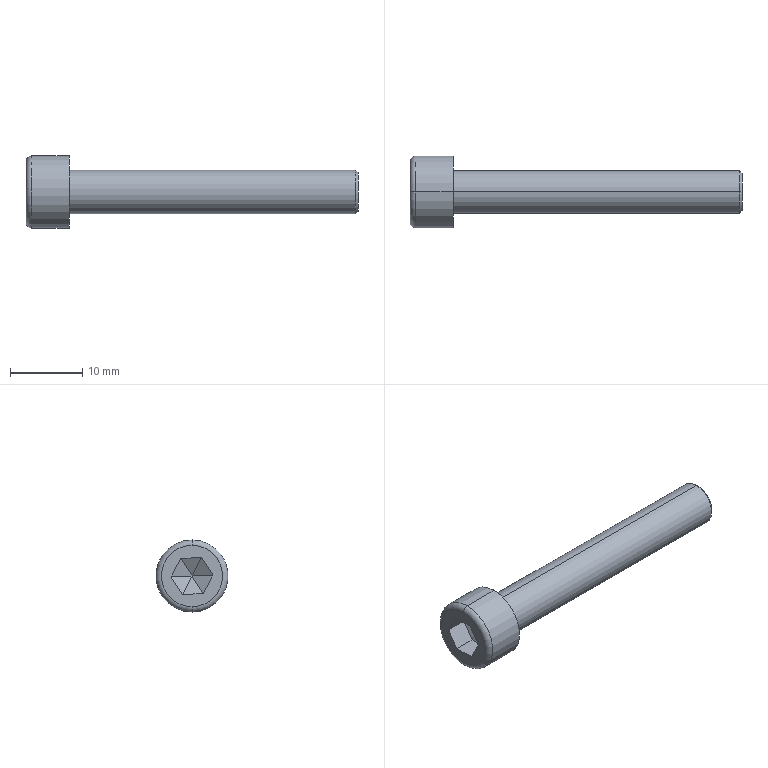Component | SolidWorks | 170423A4-ConveyorBeltIdlerAssembly1-1_170423A4-M6X40StainlessSteelCupHeadHexSocket-1 | 1 solid | 23 faces | box 46 x 10 x 10 mm | volume 1522 mm3 | plane 15 | cylinder 4 | cone 2 | torus 2 | commonest cylinder face diameters 6 x2 10 x2
STEP:
#1=CARTESIAN_POINT('',(-0.679,-3.771,17.671));
#2=VERTEX_POINT('',#1);
#3=CARTESIAN_POINT('',(-0.679,-3.771,17.88));
#4=VERTEX_POINT('',#3);
#5=CARTESIAN_POINT('',(-0.679,-3.771,17.776));
#6=DIRECTION('',(1.,0.,0.));
#7=DIRECTION('',(0.,0.,-1.));
#8=AXIS2_PLACEMENT_3D('',#5,#6,#7);
#9=CIRCLE('',#8,0.1043);
#10=EDGE_CURVE('',#2,#4,#9,.T.);
#11=ORIENTED_EDGE('',*,*,#10,.F.);
#12=CARTESIAN_POINT('',(-0.6928,-3.771,17.657));
#13=VERTEX_POINT('',#12);
#14=CARTESIAN_POINT('',(-0.679,-3.771,17.671));
#15=DIRECTION('',(-0.7071,0.,-0.7071));
#16=VECTOR('',#15,39.37);
#17=LINE('',#14,#16);
#18=EDGE_CURVE('',#2,#13,#17,.T.);
#19=ORIENTED_EDGE('',*,*,#18,.T.);
#20=CARTESIAN_POINT('',(-0.6928,-3.771,17.894));
#21=VERTEX_POINT('',#20);
#22=CARTESIAN_POINT('',(-0.6928,-3.771,17.776));
#23=DIRECTION('',(-1.,0.,0.));
#24=DIRECTION('',(0.,0.,-1.));
#25=AXIS2_PLACEMENT_3D('',#22,#23,#24);
#26=CIRCLE('',#25,0.1181);
#27=EDGE_CURVE('',#21,#13,#26,.T.);
#28=ORIENTED_EDGE('',*,*,#27,.F.);
#29=CARTESIAN_POINT('',(-0.679,-3.771,17.88));
#30=DIRECTION('',(-0.7071,0.,0.7071));
#31=VECTOR('',#30,39.37);
#32=LINE('',#29,#31);
#33=EDGE_CURVE('',#4,#21,#32,.T.);
#34=ORIENTED_EDGE('',*,*,#33,.F.);
#35=EDGE_LOOP('',(#11,#19,#28,#34));
#36=FACE_OUTER_BOUND('',#35,.T.);
#37=CARTESIAN_POINT('',(-0.679,-3.771,17.776));
#38=DIRECTION('',(-1.,0.,0.));
#39=DIRECTION('',(0.,0.,1.));
#40=AXIS2_PLACEMENT_3D('',#37,#38,#39);
#41=CONICAL_SURFACE('',#40,0.1043,0.7854);
#42=ADVANCED_FACE('',(#36),#41,.T.);
#43=CARTESIAN_POINT('',(-2.46,-3.771,17.579));
#44=VERTEX_POINT('',#43);
#45=CARTESIAN_POINT('',(-2.46,-3.771,17.972));
#46=VERTEX_POINT('',#45);
#47=CARTESIAN_POINT('',(-2.46,-3.771,17.776));
#48=DIRECTION('',(1.,0.,0.));
#49=DIRECTION('',(0.,0.,1.));
#50=AXIS2_PLACEMENT_3D('',#47,#48,#49);
#51=CIRCLE('',#50,0.1969);
#52=EDGE_CURVE('',#44,#46,#51,.T.);
#53=ORIENTED_EDGE('',*,*,#52,.F.);
#54=CARTESIAN_POINT('',(-2.49,-3.771,17.608));
#55=VERTEX_POINT('',#54);
#56=CARTESIAN_POINT('',(-2.46,-3.771,17.608));
#57=DIRECTION('',(0.,1.,0.));
#58=DIRECTION('',(0.,0.,1.));
#59=AXIS2_PLACEMENT_3D('',#56,#57,#58);
#60=CIRCLE('',#59,0.02953);
#61=EDGE_CURVE('',#44,#55,#60,.T.);
#62=ORIENTED_EDGE('',*,*,#61,.T.);
#63=CARTESIAN_POINT('',(-2.49,-3.771,17.943));
#64=VERTEX_POINT('',#63);
#65=CARTESIAN_POINT('',(-2.49,-3.771,17.776));
#66=DIRECTION('',(-1.,0.,0.));
#67=DIRECTION('',(0.,0.,1.));
#68=AXIS2_PLACEMENT_3D('',#65,#66,#67);
#69=CIRCLE('',#68,0.1673);
#70=EDGE_CURVE('',#64,#55,#69,.T.);
#71=ORIENTED_EDGE('',*,*,#70,.F.);
#72=CARTESIAN_POINT('',(-2.46,-3.771,17.943));
#73=DIRECTION('',(0.,-1.,0.));
#74=DIRECTION('',(0.,0.,-1.));
#75=AXIS2_PLACEMENT_3D('',#72,#73,#74);
#76=CIRCLE('',#75,0.02953);
#77=EDGE_CURVE('',#46,#64,#76,.T.);
#78=ORIENTED_EDGE('',*,*,#77,.F.);
#79=EDGE_LOOP('',(#53,#62,#71,#78));
#80=FACE_OUTER_BOUND('',#79,.T.);
#81=CARTESIAN_POINT('',(-2.46,-3.771,17.776));
#82=DIRECTION('',(-1.,0.,0.));
#83=DIRECTION('',(0.,0.,1.));
#84=AXIS2_PLACEMENT_3D('',#81,#82,#83);
#85=TOROIDAL_SURFACE('',#84,0.1673,0.02953);
#86=ADVANCED_FACE('',(#80),#85,.T.);
#87=ORIENTED_EDGE('',*,*,#27,.T.);
#88=CARTESIAN_POINT('',(-2.254,-3.771,17.657));
#89=VERTEX_POINT('',#88);
#90=CARTESIAN_POINT('',(-0.679,-3.771,17.657));
#91=DIRECTION('',(-1.,0.,0.));
#92=VECTOR('',#91,39.37);
#93=LINE('',#90,#92);
#94=EDGE_CURVE('',#13,#89,#93,.T.);
#95=ORIENTED_EDGE('',*,*,#94,.T.);
#96=CARTESIAN_POINT('',(-2.254,-3.771,17.894));
#97=VERTEX_POINT('',#96);
#98=CARTESIAN_POINT('',(-2.254,-3.771,17.776));
#99=DIRECTION('',(1.,0.,0.));
#100=DIRECTION('',(0.,0.,1.));
#101=AXIS2_PLACEMENT_3D('',#98,#99,#100);
#102=CIRCLE('',#101,0.1181);
#103=EDGE_CURVE('',#89,#97,#102,.T.);
#104=ORIENTED_EDGE('',*,*,#103,.T.);
#105=CARTESIAN_POINT('',(-0.679,-3.771,17.894));
#106=DIRECTION('',(-1.,0.,0.));
#107=VECTOR('',#106,39.37);
#108=LINE('',#105,#107);
#109=EDGE_CURVE('',#21,#97,#108,.T.);
#110=ORIENTED_EDGE('',*,*,#109,.F.);
#111=EDGE_LOOP('',(#87,#95,#104,#110));
#112=FACE_OUTER_BOUND('',#111,.T.);
#113=CARTESIAN_POINT('',(-0.679,-3.771,17.776));
#114=DIRECTION('',(-1.,0.,0.));
#115=DIRECTION('',(0.,0.,1.));
#116=AXIS2_PLACEMENT_3D('',#113,#114,#115);
#117=CYLINDRICAL_SURFACE('',#116,0.1181);
#118=ADVANCED_FACE('',(#112),#117,.T.);
#119=ORIENTED_EDGE('',*,*,#52,.T.);
#120=CARTESIAN_POINT('',(-2.254,-3.771,17.972));
#121=VERTEX_POINT('',#120);
#122=CARTESIAN_POINT('',(-2.49,-3.771,17.972));
#123=DIRECTION('',(1.,0.,0.));
#124=VECTOR('',#123,39.37);
#125=LINE('',#122,#124);
#126=EDGE_CURVE('',#46,#121,#125,.T.);
#127=ORIENTED_EDGE('',*,*,#126,.T.);
#128=CARTESIAN_POINT('',(-2.254,-3.771,17.579));
#129=VERTEX_POINT('',#128);
#130=CARTESIAN_POINT('',(-2.254,-3.771,17.776));
#131=DIRECTION('',(-1.,0.,0.));
#132=DIRECTION('',(0.,0.,1.));
#133=AXIS2_PLACEMENT_3D('',#130,#131,#132);
#134=CIRCLE('',#133,0.1969);
#135=EDGE_CURVE('',#121,#129,#134,.T.);
#136=ORIENTED_EDGE('',*,*,#135,.T.);
#137=CARTESIAN_POINT('',(-2.49,-3.771,17.579));
#138=DIRECTION('',(1.,0.,0.));
#139=VECTOR('',#138,39.37);
#140=LINE('',#137,#139);
#141=EDGE_CURVE('',#44,#129,#140,.T.);
#142=ORIENTED_EDGE('',*,*,#141,.F.);
#143=EDGE_LOOP('',(#119,#127,#136,#142));
#144=FACE_OUTER_BOUND('',#143,.T.);
#145=CARTESIAN_POINT('',(-2.49,-3.771,17.776));
#146=DIRECTION('',(1.,0.,0.));
#147=DIRECTION('',(0.,0.,-1.));
#148=AXIS2_PLACEMENT_3D('',#145,#146,#147);
#149=CYLINDRICAL_SURFACE('',#148,0.1969);
#150=ADVANCED_FACE('',(#144),#149,.T.);
#151=CARTESIAN_POINT('',(-2.254,-3.771,17.776));
#152=DIRECTION('',(-1.,0.,0.));
#153=DIRECTION('',(0.,0.,1.));
#154=AXIS2_PLACEMENT_3D('',#151,#152,#153);
#155=CIRCLE('',#154,0.1969);
#156=EDGE_CURVE('',#129,#121,#155,.T.);
#157=ORIENTED_EDGE('',*,*,#156,.F.);
#158=ORIENTED_EDGE('',*,*,#135,.F.);
#159=EDGE_LOOP('',(#157,#158));
#160=FACE_OUTER_BOUND('',#159,.T.);
#161=CARTESIAN_POINT('',(-2.254,-3.771,17.776));
#162=DIRECTION('',(1.,0.,0.));
#163=DIRECTION('',(0.,0.,1.));
#164=AXIS2_PLACEMENT_3D('',#161,#162,#163);
#165=CIRCLE('',#164,0.1181);
#166=EDGE_CURVE('',#97,#89,#165,.T.);
#167=ORIENTED_EDGE('',*,*,#166,.F.);
#168=ORIENTED_EDGE('',*,*,#103,.F.);
#169=EDGE_LOOP('',(#167,#168));
#170=FACE_BOUND('',#169,.T.);
#171=CARTESIAN_POINT('',(-2.254,-3.771,17.776));
#172=DIRECTION('',(-1.,0.,0.));
#173=DIRECTION('',(0.,0.,1.));
#174=AXIS2_PLACEMENT_3D('',#171,#172,#173);
#175=PLANE('',#174);
#176=ADVANCED_FACE('',(#160,#170),#175,.F.);
#177=ORIENTED_EDGE('',*,*,#126,.F.);
#178=CARTESIAN_POINT('',(-2.46,-3.771,17.776));
#179=DIRECTION('',(1.,0.,0.));
#180=DIRECTION('',(0.,0.,1.));
#181=AXIS2_PLACEMENT_3D('',#178,#179,#180);
#182=CIRCLE('',#181,0.1969);
#183=EDGE_CURVE('',#46,#44,#182,.T.);
#184=ORIENTED_EDGE('',*,*,#183,.T.);
#185=ORIENTED_EDGE('',*,*,#141,.T.);
#186=ORIENTED_EDGE('',*,*,#156,.T.);
#187=EDGE_LOOP('',(#177,#184,#185,#186));
#188=FACE_OUTER_BOUND('',#187,.T.);
#189=CARTESIAN_POINT('',(-2.49,-3.771,17.776));
#190=DIRECTION('',(1.,0.,0.));
#191=DIRECTION('',(0.,0.,-1.));
#192=AXIS2_PLACEMENT_3D('',#189,#190,#191);
#193=CYLINDRICAL_SURFACE('',#192,0.1969);
#194=ADVANCED_FACE('',(#188),#193,.T.);
#195=ORIENTED_EDGE('',*,*,#70,.T.);
#196=CARTESIAN_POINT('',(-2.49,-3.771,17.776));
#197=DIRECTION('',(-1.,0.,0.));
#198=DIRECTION('',(0.,0.,1.));
#199=AXIS2_PLACEMENT_3D('',#196,#197,#198);
#200=CIRCLE('',#199,0.1673);
#201=EDGE_CURVE('',#55,#64,#200,.T.);
#202=ORIENTED_EDGE('',*,*,#201,.T.);
#203=EDGE_LOOP('',(#195,#202));
#204=FACE_OUTER_BOUND('',#203,.T.);
#205=CARTESIAN_POINT('',(-2.49,-3.833,17.68));
#206=VERTEX_POINT('',#205);
#207=CARTESIAN_POINT('',(-2.49,-3.885,17.781));
#208=VERTEX_POINT('',#207);
#209=CARTESIAN_POINT('',(-2.49,-3.833,17.68));
#210=DIRECTION('',(0.,-0.4558,0.8901));
#211=VECTOR('',#210,39.37);
#212=LINE('',#209,#211);
#213=EDGE_CURVE('',#206,#208,#212,.T.);
#214=ORIENTED_EDGE('',*,*,#213,.F.);
#215=CARTESIAN_POINT('',(-2.49,-3.719,17.674));
#216=VERTEX_POINT('',#215);
#217=CARTESIAN_POINT('',(-2.49,-3.719,17.674));
#218=DIRECTION('',(0.,-0.9987,0.05033));
#219=VECTOR('',#218,39.37);
#220=LINE('',#217,#219);
#221=EDGE_CURVE('',#216,#206,#220,.T.);
#222=ORIENTED_EDGE('',*,*,#221,.F.);
#223=CARTESIAN_POINT('',(-2.49,-3.658,17.77));
#224=VERTEX_POINT('',#223);
#225=CARTESIAN_POINT('',(-2.49,-3.658,17.77));
#226=DIRECTION('',(0.,-0.543,-0.8398));
#227=VECTOR('',#226,39.37);
#228=LINE('',#225,#227);
#229=EDGE_CURVE('',#224,#216,#228,.T.);
#230=ORIENTED_EDGE('',*,*,#229,.F.);
#231=CARTESIAN_POINT('',(-2.49,-3.709,17.871));
#232=VERTEX_POINT('',#231);
#233=CARTESIAN_POINT('',(-2.49,-3.709,17.871));
#234=DIRECTION('',(0.,0.4558,-0.8901));
#235=VECTOR('',#234,39.37);
#236=LINE('',#233,#235);
#237=EDGE_CURVE('',#232,#224,#236,.T.);
#238=ORIENTED_EDGE('',*,*,#237,.F.);
#239=CARTESIAN_POINT('',(-2.49,-3.823,17.877));
#240=VERTEX_POINT('',#239);
#241=CARTESIAN_POINT('',(-2.49,-3.823,17.877));
#242=DIRECTION('',(0.,0.9987,-0.05033));
#243=VECTOR('',#242,39.37);
#244=LINE('',#241,#243);
#245=EDGE_CURVE('',#240,#232,#244,.T.);
#246=ORIENTED_EDGE('',*,*,#245,.F.);
#247=CARTESIAN_POINT('',(-2.49,-3.885,17.781));
#248=DIRECTION('',(0.,0.543,0.8398));
#249=VECTOR('',#248,39.37);
#250=LINE('',#247,#249);
#251=EDGE_CURVE('',#208,#240,#250,.T.);
#252=ORIENTED_EDGE('',*,*,#251,.F.);
#253=EDGE_LOOP('',(#214,#222,#230,#238,#246,#252));
#254=FACE_BOUND('',#253,.T.);
#255=CARTESIAN_POINT('',(-2.49,-3.771,17.776));
#256=DIRECTION('',(-1.,0.,0.));
#257=DIRECTION('',(0.,0.,1.));
#258=AXIS2_PLACEMENT_3D('',#255,#256,#257);
#259=PLANE('',#258);
#260=ADVANCED_FACE('',(#204,#254),#259,.T.);
#261=ORIENTED_EDGE('',*,*,#213,.T.);
#262=CARTESIAN_POINT('',(-2.372,-3.885,17.781));
#263=VERTEX_POINT('',#262);
#264=CARTESIAN_POINT('',(-2.372,-3.885,17.781));
#265=DIRECTION('',(-1.,0.,0.));
#266=VECTOR('',#265,39.37);
#267=LINE('',#264,#266);
#268=EDGE_CURVE('',#263,#208,#267,.T.);
#269=ORIENTED_EDGE('',*,*,#268,.F.);
#270=CARTESIAN_POINT('',(-2.372,-3.833,17.68));
#271=VERTEX_POINT('',#270);
#272=CARTESIAN_POINT('',(-2.372,-3.833,17.68));
#273=DIRECTION('',(0.,-0.4558,0.8901));
#274=VECTOR('',#273,39.37);
#275=LINE('',#272,#274);
#276=EDGE_CURVE('',#271,#263,#275,.T.);
#277=ORIENTED_EDGE('',*,*,#276,.F.);
#278=CARTESIAN_POINT('',(-2.372,-3.833,17.68));
#279=DIRECTION('',(-1.,0.,0.));
#280=VECTOR('',#279,39.37);
#281=LINE('',#278,#280);
#282=EDGE_CURVE('',#271,#206,#281,.T.);
#283=ORIENTED_EDGE('',*,*,#282,.T.);
#284=EDGE_LOOP('',(#261,#269,#277,#283));
#285=FACE_OUTER_BOUND('',#284,.T.);
#286=CARTESIAN_POINT('',(-2.372,-3.833,17.68));
#287=DIRECTION('',(0.,-0.8901,-0.4558));
#288=DIRECTION('',(0.,-0.4558,0.8901));
#289=AXIS2_PLACEMENT_3D('',#286,#287,#288);
#290=PLANE('',#289);
#291=ADVANCED_FACE('',(#285),#290,.F.);
#292=ORIENTED_EDGE('',*,*,#221,.T.);
#293=ORIENTED_EDGE('',*,*,#282,.F.);
#294=CARTESIAN_POINT('',(-2.372,-3.719,17.674));
#295=VERTEX_POINT('',#294);
#296=CARTESIAN_POINT('',(-2.372,-3.719,17.674));
#297=DIRECTION('',(0.,-0.9987,0.05033));
#298=VECTOR('',#297,39.37);
#299=LINE('',#296,#298);
#300=EDGE_CURVE('',#295,#271,#299,.T.);
#301=ORIENTED_EDGE('',*,*,#300,.F.);
#302=CARTESIAN_POINT('',(-2.372,-3.719,17.674));
#303=DIRECTION('',(-1.,0.,0.));
#304=VECTOR('',#303,39.37);
#305=LINE('',#302,#304);
#306=EDGE_CURVE('',#295,#216,#305,.T.);
#307=ORIENTED_EDGE('',*,*,#306,.T.);
#308=EDGE_LOOP('',(#292,#293,#301,#307));
#309=FACE_OUTER_BOUND('',#308,.T.);
#310=CARTESIAN_POINT('',(-2.372,-3.719,17.674));
#311=DIRECTION('',(0.,-0.05033,-0.9987));
#312=DIRECTION('',(0.,-0.9987,0.05033));
#313=AXIS2_PLACEMENT_3D('',#310,#311,#312);
#314=PLANE('',#313);
#315=ADVANCED_FACE('',(#309),#314,.F.);
#316=ORIENTED_EDGE('',*,*,#229,.T.);
#317=ORIENTED_EDGE('',*,*,#306,.F.);
#318=CARTESIAN_POINT('',(-2.372,-3.658,17.77));
#319=VERTEX_POINT('',#318);
#320=CARTESIAN_POINT('',(-2.372,-3.658,17.77));
#321=DIRECTION('',(0.,-0.543,-0.8398));
#322=VECTOR('',#321,39.37);
#323=LINE('',#320,#322);
#324=EDGE_CURVE('',#319,#295,#323,.T.);
#325=ORIENTED_EDGE('',*,*,#324,.F.);
#326=CARTESIAN_POINT('',(-2.372,-3.658,17.77));
#327=DIRECTION('',(-1.,0.,0.));
#328=VECTOR('',#327,39.37);
#329=LINE('',#326,#328);
#330=EDGE_CURVE('',#319,#224,#329,.T.);
#331=ORIENTED_EDGE('',*,*,#330,.T.);
#332=EDGE_LOOP('',(#316,#317,#325,#331));
#333=FACE_OUTER_BOUND('',#332,.T.);
#334=CARTESIAN_POINT('',(-2.372,-3.658,17.77));
#335=DIRECTION('',(0.,0.8398,-0.543));
#336=DIRECTION('',(0.,-0.543,-0.8398));
#337=AXIS2_PLACEMENT_3D('',#334,#335,#336);
#338=PLANE('',#337);
#339=ADVANCED_FACE('',(#333),#338,.F.);
#340=ORIENTED_EDGE('',*,*,#237,.T.);
#341=ORIENTED_EDGE('',*,*,#330,.F.);
#342=CARTESIAN_POINT('',(-2.372,-3.709,17.871));
#343=VERTEX_POINT('',#342);
#344=CARTESIAN_POINT('',(-2.372,-3.709,17.871));
#345=DIRECTION('',(0.,0.4558,-0.8901));
#346=VECTOR('',#345,39.37);
#347=LINE('',#344,#346);
#348=EDGE_CURVE('',#343,#319,#347,.T.);
#349=ORIENTED_EDGE('',*,*,#348,.F.);
#350=CARTESIAN_POINT('',(-2.372,-3.709,17.871));
#351=DIRECTION('',(-1.,0.,0.));
#352=VECTOR('',#351,39.37);
#353=LINE('',#350,#352);
#354=EDGE_CURVE('',#343,#232,#353,.T.);
#355=ORIENTED_EDGE('',*,*,#354,.T.);
#356=EDGE_LOOP('',(#340,#341,#349,#355));
#357=FACE_OUTER_BOUND('',#356,.T.);
#358=CARTESIAN_POINT('',(-2.372,-3.709,17.871));
#359=DIRECTION('',(0.,0.8901,0.4558));
#360=DIRECTION('',(0.,0.4558,-0.8901));
#361=AXIS2_PLACEMENT_3D('',#358,#359,#360);
#362=PLANE('',#361);
#363=ADVANCED_FACE('',(#357),#362,.F.);
#364=ORIENTED_EDGE('',*,*,#245,.T.);
#365=ORIENTED_EDGE('',*,*,#354,.F.);
#366=CARTESIAN_POINT('',(-2.372,-3.823,17.877));
#367=VERTEX_POINT('',#366);
#368=CARTESIAN_POINT('',(-2.372,-3.823,17.877));
#369=DIRECTION('',(0.,0.9987,-0.05033));
#370=VECTOR('',#369,39.37);
#371=LINE('',#368,#370);
#372=EDGE_CURVE('',#367,#343,#371,.T.);
#373=ORIENTED_EDGE('',*,*,#372,.F.);
#374=CARTESIAN_POINT('',(-2.372,-3.823,17.877));
#375=DIRECTION('',(-1.,0.,0.));
#376=VECTOR('',#375,39.37);
#377=LINE('',#374,#376);
#378=EDGE_CURVE('',#367,#240,#377,.T.);
#379=ORIENTED_EDGE('',*,*,#378,.T.);
#380=EDGE_LOOP('',(#364,#365,#373,#379));
#381=FACE_OUTER_BOUND('',#380,.T.);
#382=CARTESIAN_POINT('',(-2.372,-3.823,17.877));
#383=DIRECTION('',(0.,0.05033,0.9987));
#384=DIRECTION('',(0.,0.9987,-0.05033));
#385=AXIS2_PLACEMENT_3D('',#382,#383,#384);
#386=PLANE('',#385);
#387=ADVANCED_FACE('',(#381),#386,.F.);
#388=ORIENTED_EDGE('',*,*,#251,.T.);
#389=ORIENTED_EDGE('',*,*,#378,.F.);
#390=CARTESIAN_POINT('',(-2.372,-3.885,17.781));
#391=DIRECTION('',(0.,0.543,0.8398));
#392=VECTOR('',#391,39.37);
#393=LINE('',#390,#392);
#394=EDGE_CURVE('',#263,#367,#393,.T.);
#395=ORIENTED_EDGE('',*,*,#394,.F.);
#396=ORIENTED_EDGE('',*,*,#268,.T.);
#397=EDGE_LOOP('',(#388,#389,#395,#396));
#398=FACE_OUTER_BOUND('',#397,.T.);
#399=CARTESIAN_POINT('',(-2.372,-3.885,17.781));
#400=DIRECTION('',(0.,-0.8398,0.543));
#401=DIRECTION('',(0.,0.543,0.8398));
#402=AXIS2_PLACEMENT_3D('',#399,#400,#401);
#403=PLANE('',#402);
#404=ADVANCED_FACE('',(#398),#403,.F.);
#405=ORIENTED_EDGE('',*,*,#94,.F.);
#406=CARTESIAN_POINT('',(-0.6928,-3.771,17.776));
#407=DIRECTION('',(-1.,0.,0.));
#408=DIRECTION('',(0.,0.,-1.));
#409=AXIS2_PLACEMENT_3D('',#406,#407,#408);
#410=CIRCLE('',#409,0.1181);
#411=EDGE_CURVE('',#13,#21,#410,.T.);
#412=ORIENTED_EDGE('',*,*,#411,.T.);
#413=ORIENTED_EDGE('',*,*,#109,.T.);
#414=ORIENTED_EDGE('',*,*,#166,.T.);
#415=EDGE_LOOP('',(#405,#412,#413,#414));
#416=FACE_OUTER_BOUND('',#415,.T.);
#417=CARTESIAN_POINT('',(-0.679,-3.771,17.776));
#418=DIRECTION('',(-1.,0.,0.));
#419=DIRECTION('',(0.,0.,1.));
#420=AXIS2_PLACEMENT_3D('',#417,#418,#419);
#421=CYLINDRICAL_SURFACE('',#420,0.1181);
#422=ADVANCED_FACE('',(#416),#421,.T.);
#423=CARTESIAN_POINT('',(-0.679,-3.771,17.776));
#424=DIRECTION('',(1.,0.,0.));
#425=DIRECTION('',(0.,0.,-1.));
#426=AXIS2_PLACEMENT_3D('',#423,#424,#425);
#427=CIRCLE('',#426,0.1043);
#428=EDGE_CURVE('',#4,#2,#427,.T.);
#429=ORIENTED_EDGE('',*,*,#428,.T.);
#430=ORIENTED_EDGE('',*,*,#10,.T.);
#431=EDGE_LOOP('',(#429,#430));
#432=FACE_OUTER_BOUND('',#431,.T.);
#433=CARTESIAN_POINT('',(-0.679,-3.771,17.776));
#434=DIRECTION('',(1.,0.,0.));
#435=DIRECTION('',(0.,0.,-1.));
#436=AXIS2_PLACEMENT_3D('',#433,#434,#435);
#437=PLANE('',#436);
#438=ADVANCED_FACE('',(#432),#437,.T.);
#439=ORIENTED_EDGE('',*,*,#348,.T.);
#440=CARTESIAN_POINT('',(-2.315,-3.771,17.776));
#441=VERTEX_POINT('',#440);
#442=CARTESIAN_POINT('',(-2.349,-3.703,17.772));
#443=DIRECTION('',(-0.4472,0.8933,-0.04502));
#444=VECTOR('',#443,39.37);
#445=LINE('',#442,#444);
#446=EDGE_CURVE('',#441,#319,#445,.T.);
#447=ORIENTED_EDGE('',*,*,#446,.F.);
#448=CARTESIAN_POINT('',(-2.349,-3.734,17.833));
#449=DIRECTION('',(-0.4472,0.4856,0.7511));
#450=VECTOR('',#449,39.37);
#451=LINE('',#448,#450);
#452=EDGE_CURVE('',#441,#343,#451,.T.);
#453=ORIENTED_EDGE('',*,*,#452,.T.);
#454=EDGE_LOOP('',(#439,#447,#453));
#455=FACE_OUTER_BOUND('',#454,.T.);
#456=CARTESIAN_POINT('',(-2.372,-3.709,17.871));
#457=DIRECTION('',(0.866,0.445,0.2279));
#458=DIRECTION('',(-0.4571,0.8894,0.));
#459=AXIS2_PLACEMENT_3D('',#456,#457,#458);
#460=PLANE('',#459);
#461=ADVANCED_FACE('',(#455),#460,.F.);
#462=ORIENTED_EDGE('',*,*,#372,.T.);
#463=ORIENTED_EDGE('',*,*,#452,.F.);
#464=CARTESIAN_POINT('',(-2.349,-3.802,17.836));
#465=DIRECTION('',(-0.4472,-0.4077,0.7961));
#466=VECTOR('',#465,39.37);
#467=LINE('',#464,#466);
#468=EDGE_CURVE('',#441,#367,#467,.T.);
#469=ORIENTED_EDGE('',*,*,#468,.T.);
#470=EDGE_LOOP('',(#462,#463,#469));
#471=FACE_OUTER_BOUND('',#470,.T.);
#472=CARTESIAN_POINT('',(-2.372,-3.823,17.877));
#473=DIRECTION('',(0.866,0.02517,0.4994));
#474=DIRECTION('',(0.4995,0.,-0.8663));
#475=AXIS2_PLACEMENT_3D('',#472,#473,#474);
#476=PLANE('',#475);
#477=ADVANCED_FACE('',(#471),#476,.F.);
#478=ORIENTED_EDGE('',*,*,#394,.T.);
#479=ORIENTED_EDGE('',*,*,#468,.F.);
#480=CARTESIAN_POINT('',(-2.349,-3.839,17.779));
#481=DIRECTION('',(-0.4472,-0.8933,0.04502));
#482=VECTOR('',#481,39.37);
#483=LINE('',#480,#482);
#484=EDGE_CURVE('',#441,#263,#483,.T.);
#485=ORIENTED_EDGE('',*,*,#484,.T.);
#486=EDGE_LOOP('',(#478,#479,#485));
#487=FACE_OUTER_BOUND('',#486,.T.);
#488=CARTESIAN_POINT('',(-2.372,-3.885,17.781));
#489=DIRECTION('',(0.866,-0.4199,0.2715));
#490=DIRECTION('',(0.4363,0.8998,0.));
#491=AXIS2_PLACEMENT_3D('',#488,#489,#490);
#492=PLANE('',#491);
#493=ADVANCED_FACE('',(#487),#492,.F.);
#494=ORIENTED_EDGE('',*,*,#276,.T.);
#495=ORIENTED_EDGE('',*,*,#484,.F.);
#496=CARTESIAN_POINT('',(-2.349,-3.808,17.718));
#497=DIRECTION('',(-0.4472,-0.4856,-0.7511));
#498=VECTOR('',#497,39.37);
#499=LINE('',#496,#498);
#500=EDGE_CURVE('',#441,#271,#499,.T.);
#501=ORIENTED_EDGE('',*,*,#500,.T.);
#502=EDGE_LOOP('',(#494,#495,#501));
#503=FACE_OUTER_BOUND('',#502,.T.);
#504=CARTESIAN_POINT('',(-2.372,-3.833,17.68));
#505=DIRECTION('',(0.866,-0.445,-0.2279));
#506=DIRECTION('',(0.4571,0.8894,0.));
#507=AXIS2_PLACEMENT_3D('',#504,#505,#506);
#508=PLANE('',#507);
#509=ADVANCED_FACE('',(#503),#508,.F.);
#510=ORIENTED_EDGE('',*,*,#300,.T.);
#511=ORIENTED_EDGE('',*,*,#500,.F.);
#512=CARTESIAN_POINT('',(-2.349,-3.74,17.715));
#513=DIRECTION('',(-0.4472,0.4077,-0.7961));
#514=VECTOR('',#513,39.37);
#515=LINE('',#512,#514);
#516=EDGE_CURVE('',#441,#295,#515,.T.);
#517=ORIENTED_EDGE('',*,*,#516,.T.);
#518=EDGE_LOOP('',(#510,#511,#517));
#519=FACE_OUTER_BOUND('',#518,.T.);
#520=CARTESIAN_POINT('',(-2.372,-3.719,17.674));
#521=DIRECTION('',(0.866,-0.02517,-0.4994));
#522=DIRECTION('',(-0.4995,0.,-0.8663));
#523=AXIS2_PLACEMENT_3D('',#520,#521,#522);
#524=PLANE('',#523);
#525=ADVANCED_FACE('',(#519),#524,.F.);
#526=ORIENTED_EDGE('',*,*,#324,.T.);
#527=ORIENTED_EDGE('',*,*,#516,.F.);
#528=ORIENTED_EDGE('',*,*,#446,.T.);
#529=EDGE_LOOP('',(#526,#527,#528));
#530=FACE_OUTER_BOUND('',#529,.T.);
#531=CARTESIAN_POINT('',(-2.372,-3.658,17.77));
#532=DIRECTION('',(0.866,0.4199,-0.2715));
#533=DIRECTION('',(-0.4363,0.8998,0.));
#534=AXIS2_PLACEMENT_3D('',#531,#532,#533);
#535=PLANE('',#534);
#536=ADVANCED_FACE('',(#530),#535,.F.);
#537=ORIENTED_EDGE('',*,*,#61,.F.);
#538=ORIENTED_EDGE('',*,*,#183,.F.);
#539=ORIENTED_EDGE('',*,*,#77,.T.);
#540=ORIENTED_EDGE('',*,*,#201,.F.);
#541=EDGE_LOOP('',(#537,#538,#539,#540));
#542=FACE_OUTER_BOUND('',#541,.T.);
#543=CARTESIAN_POINT('',(-2.46,-3.771,17.776));
#544=DIRECTION('',(-1.,0.,0.));
#545=DIRECTION('',(0.,0.,1.));
#546=AXIS2_PLACEMENT_3D('',#543,#544,#545);
#547=TOROIDAL_SURFACE('',#546,0.1673,0.02953);
#548=ADVANCED_FACE('',(#542),#547,.T.);
#549=ORIENTED_EDGE('',*,*,#18,.F.);
#550=ORIENTED_EDGE('',*,*,#428,.F.);
#551=ORIENTED_EDGE('',*,*,#33,.T.);
#552=ORIENTED_EDGE('',*,*,#411,.F.);
#553=EDGE_LOOP('',(#549,#550,#551,#552));
#554=FACE_OUTER_BOUND('',#553,.T.);
#555=CARTESIAN_POINT('',(-0.679,-3.771,17.776));
#556=DIRECTION('',(-1.,0.,0.));
#557=DIRECTION('',(0.,0.,1.));
#558=AXIS2_PLACEMENT_3D('',#555,#556,#557);
#559=CONICAL_SURFACE('',#558,0.1043,0.7854);
#560=ADVANCED_FACE('',(#554),#559,.T.);
#561=CLOSED_SHELL('',(#42,#86,#118,#150,#176,#194,#260,#291,#315,#339,#363,#387,#404,#422,#438,#461,#477,#493,#509,#525,#536,#548,#560));
#562=MANIFOLD_SOLID_BREP('',#561);
#563=CARTESIAN_POINT('',(0.,0.,0.));
#564=DIRECTION('',(0.,0.,1.));
#565=DIRECTION('',(1.,0.,0.));
#566=AXIS2_PLACEMENT_3D('',#563,#564,#565);
#567=(LENGTH_UNIT()NAMED_UNIT(*)SI_UNIT($,.METRE.));
#568=LENGTH_MEASURE_WITH_UNIT(LENGTH_MEASURE(0.0254),#567);
#569=DIMENSIONAL_EXPONENTS(1.,0.,0.,0.,0.,0.,0.);
#570=(CONVERSION_BASED_UNIT('',#568)LENGTH_UNIT()NAMED_UNIT(#569));
#571=UNCERTAINTY_MEASURE_WITH_UNIT(LENGTH_MEASURE(0.00001),#570,'','');
#572=(NAMED_UNIT(*)PLANE_ANGLE_UNIT()SI_UNIT($,.RADIAN.));
#573=(NAMED_UNIT(*)SI_UNIT($,.STERADIAN.)SOLID_ANGLE_UNIT());
#574=(GEOMETRIC_REPRESENTATION_CONTEXT(3)GLOBAL_UNCERTAINTY_ASSIGNED_CONTEXT((#571))GLOBAL_UNIT_ASSIGNED_CONTEXT((#570,#572,#573))REPRESENTATION_CONTEXT('',''));
#575=ADVANCED_BREP_SHAPE_REPRESENTATION('',(#562,#566),#574);
#576=COLOUR_RGB('',0.7922,0.8196,0.9333);
#577=FILL_AREA_STYLE_COLOUR('',#576);
#578=FILL_AREA_STYLE('',(#577));
#579=SURFACE_STYLE_FILL_AREA(#578);
#580=SURFACE_SIDE_STYLE('',(#579));
#581=SURFACE_STYLE_USAGE(.BOTH.,#580);
#582=PRESENTATION_STYLE_ASSIGNMENT((#581));
#583=STYLED_ITEM('',(#582),#562);
#584=PRESENTATION_LAYER_ASSIGNMENT('','',(#583));
#585=(LENGTH_UNIT()NAMED_UNIT(*)SI_UNIT($,.METRE.));
#586=LENGTH_MEASURE_WITH_UNIT(LENGTH_MEASURE(0.0254),#585);
#587=DIMENSIONAL_EXPONENTS(1.,0.,0.,0.,0.,0.,0.);
#588=(CONVERSION_BASED_UNIT('',#586)LENGTH_UNIT()NAMED_UNIT(#587));
#589=UNCERTAINTY_MEASURE_WITH_UNIT(LENGTH_MEASURE(0.00001),#588,'','');
#590=(NAMED_UNIT(*)PLANE_ANGLE_UNIT()SI_UNIT($,.RADIAN.));
#591=(NAMED_UNIT(*)SI_UNIT($,.STERADIAN.)SOLID_ANGLE_UNIT());
#592=(GEOMETRIC_REPRESENTATION_CONTEXT(3)GLOBAL_UNCERTAINTY_ASSIGNED_CONTEXT((#589))GLOBAL_UNIT_ASSIGNED_CONTEXT((#588,#590,#591))REPRESENTATION_CONTEXT('',''));
#593=MECHANICAL_DESIGN_GEOMETRIC_PRESENTATION_REPRESENTATION('',(#583),#592);